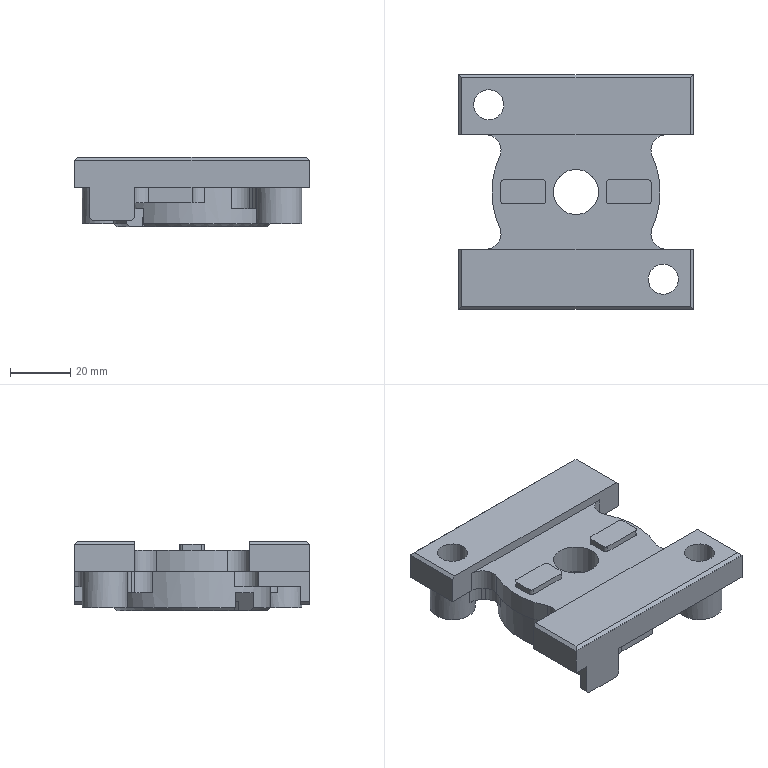CAM job | NX | mm | 3-axis | 2 set-ups | 21 operations | part box 78 x 78 x 23
set-up 1
1. Volume Based 2.5D Milling | Mill Mill5 D10 | FLOOR_WALL | path 1100.537 mm | 0.7224 min
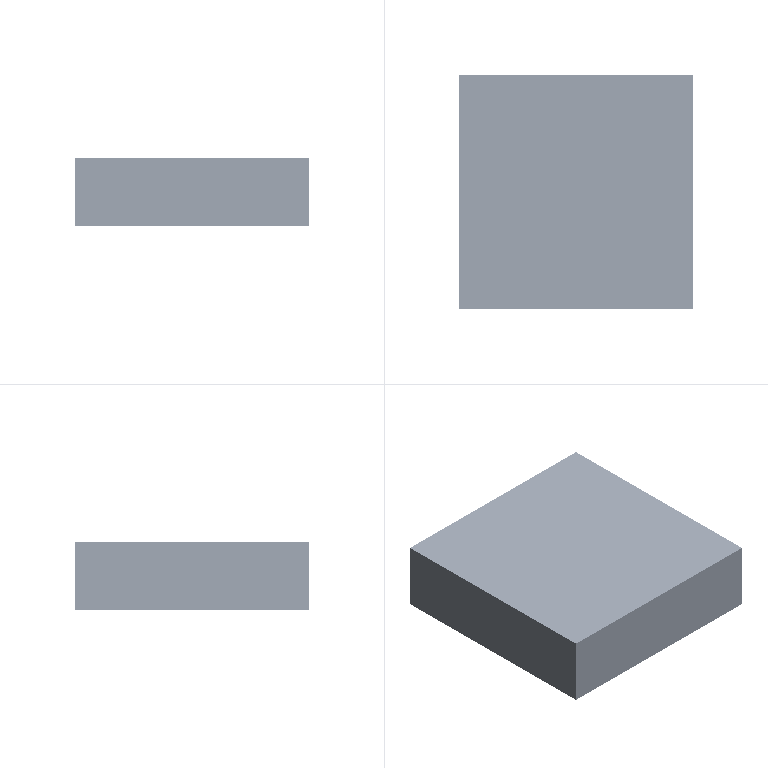2. Adaptive Milling | Mill Mill5 D10 | ADAPTIVE_MILLING | path 2222.462 mm | 1.684 min
3. Cavity Milling | Mill Mill5 D10 | CAVITY_MILL | path 2178.169 mm | 1.458 min
4. Volume Based 2.5D Milling | Mill Mill5 D10 | FLOOR_WALL_1 | path 353.649 mm | 0.2786 min
5. Volume Based 2.5D Milling | Mill Mill5 D10 | FLOOR_WALL_2 | path 207.012 mm | 0.1173 min
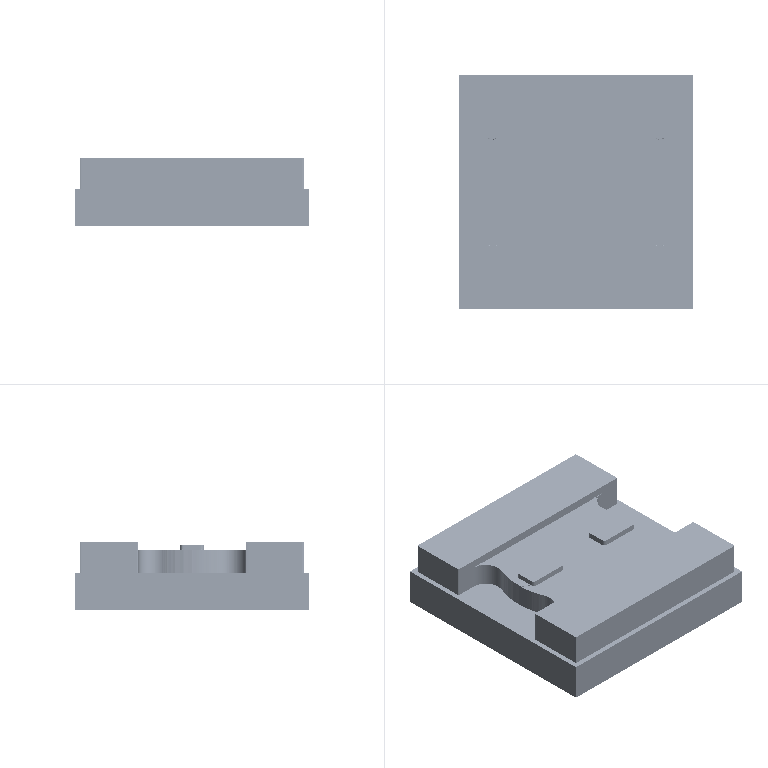6. Planar Milling | Mill Mill5 D10 | PLANAR_PROFILE | path 249.186 mm | 0.1622 min
7. Planar Milling | Mill Mill5 D10 | PLANAR_PROFILE_1 | path 264.815 mm | 0.1851 min
8. Volume Based 2.5D Milling | Mill Mill5 D10 | FLOOR_WALL_3 | path 702.548 mm | 0.482 min
9. Planar Milling | Mill Mill5 D10 | PLANAR_PROFILE_2 | path 445.502 mm | 0.3449 min
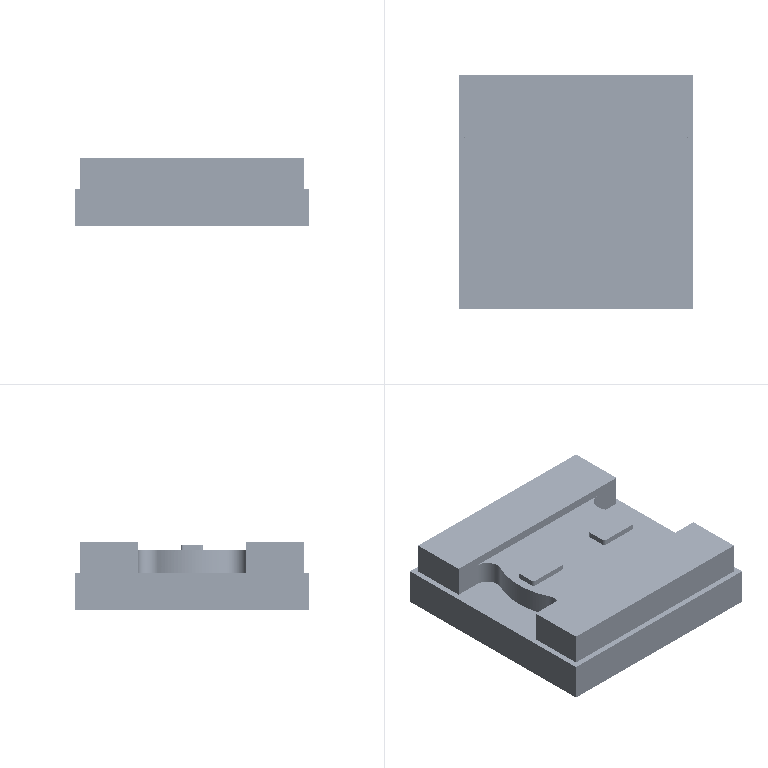10. Cylinder Milling | Mill Mill5 D10 | HOLE_MILLING | path 658.16 mm | 0.8729 min
11. Cylinder Milling | Mill Mill5 D10 | HOLE_MILLING_COPY | path 130.04 mm | 0.3453 min
12. Cylinder Milling | Mill Mill5 D6 | HOLE_MILLING_1 | path 1540.137 mm | 1.973 min
13. Cylinder Milling | Mill Mill5 D6 | HOLE_MILLING_1_COPY | path 285.883 mm | 0.4459 min
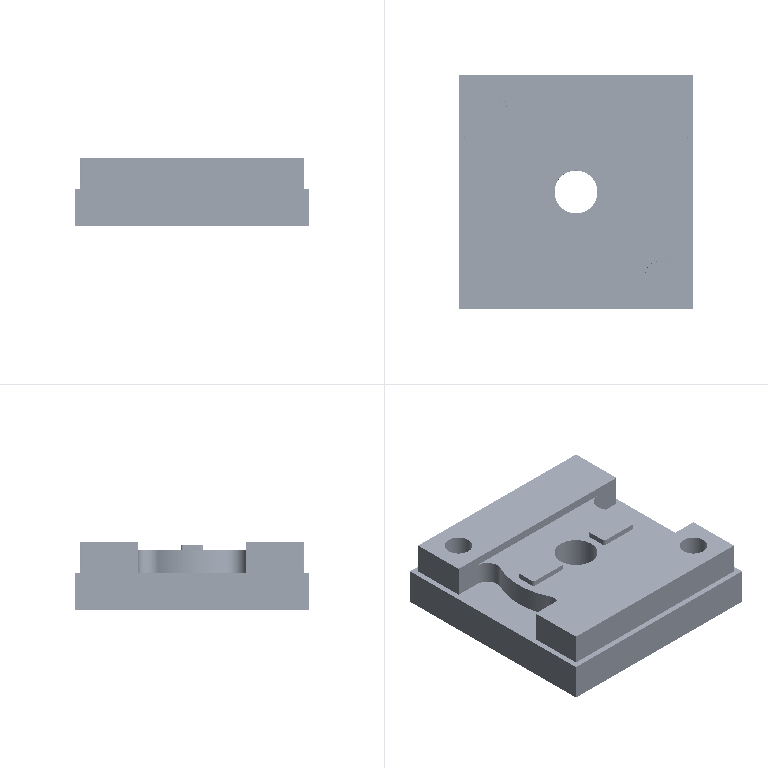14. Planar Milling | Mill Mill5 D6 | SOLID_PROFILE_3D | path 346.274 mm | 0.2372 min
set-up 2
15. Volume Based 2.5D Milling | Mill Mill5 D10 | FLOOR_WALL_4 | path 1100.644 mm | 0.8333 min
16. Adaptive Milling | Mill Mill5 D10 | ADAPTIVE_MILLING_1 | path 5745.657 mm | 3.944 min
17. Adaptive Milling | Mill Mill5 D10 | ADAPTIVE_MILLING_1_COPY | path 2146.8 mm | 1.311 min
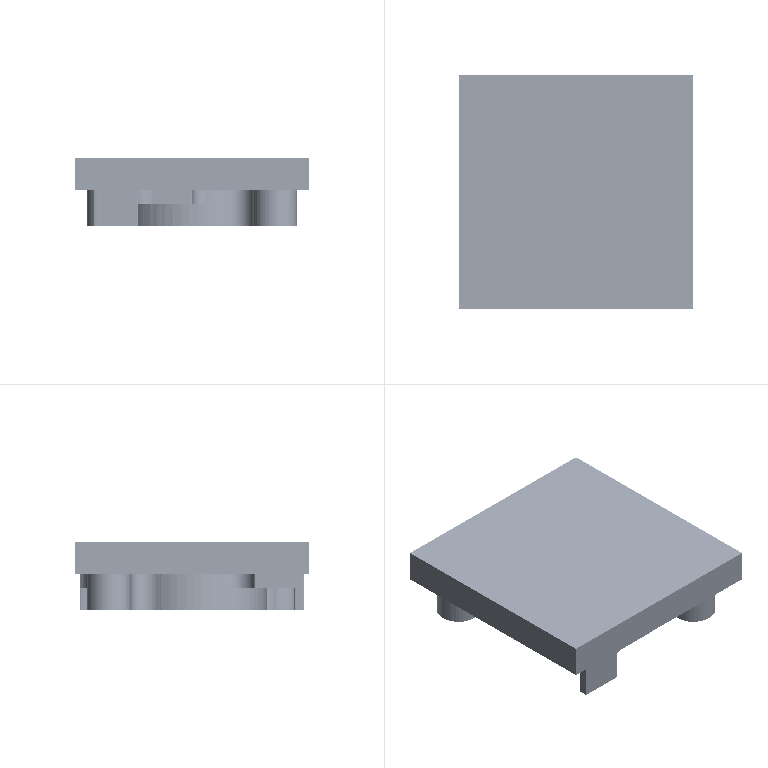18. Adaptive Milling | Mill Mill5 D10 | ADAPTIVE_MILLING_1_COPY_COPY | path 303.515 mm | 0.1124 min
19. Adaptive Milling | Mill Mill5 D10 | ADAPTIVE_MILLING_1_COPY_COPY_COPY | path 679.913 mm | 0.4734 min
20. Adaptive Milling | Mill Mill5 D10 | ADAPTIVE_MILLING_1_COPY_COPY_COPY_COPY | path 207.935 mm | 0.07878 min
21. Adaptive Milling | Mill Mill5 D10 | ADAPTIVE_MILLING_1_COPY_COPY_COPY_COPY_COPY | path 1086.929 mm | 0.6379 min